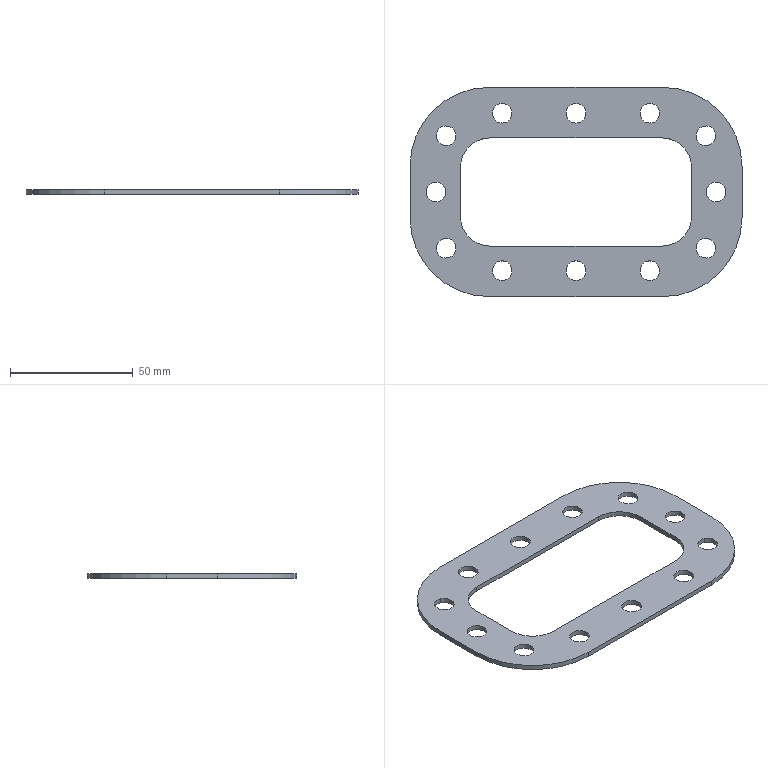Component | NX | WASHER | 1 solid | 34 faces | volume 11960 mm3 | cylinder 24 | plane 10 | commonest cylinder face diameters 8 x16 64 x4 24 x4